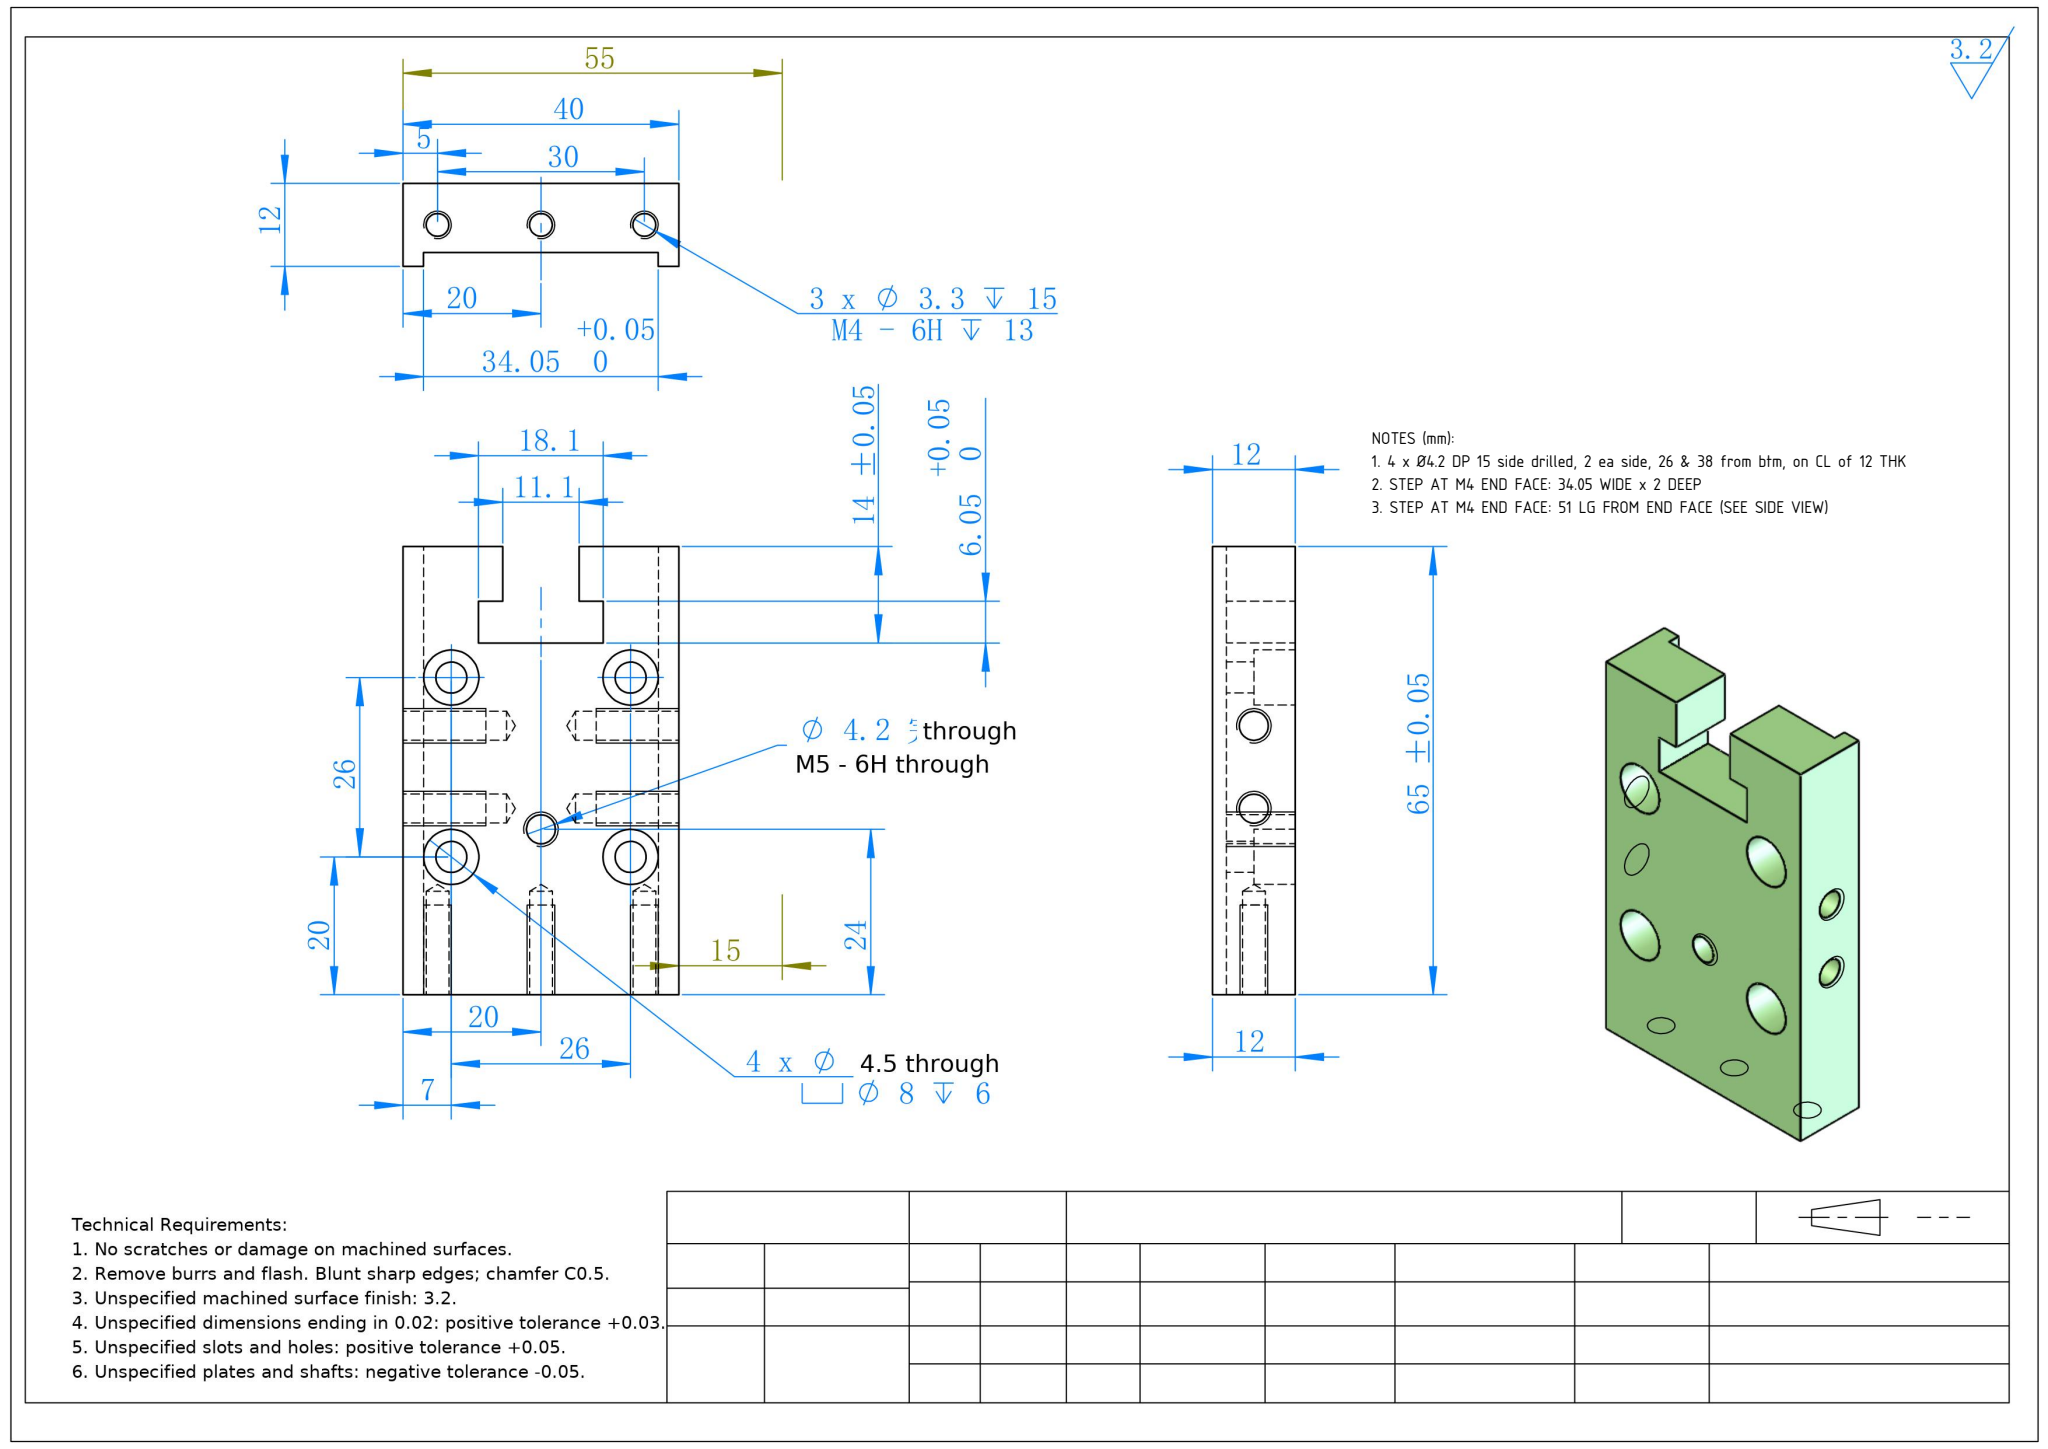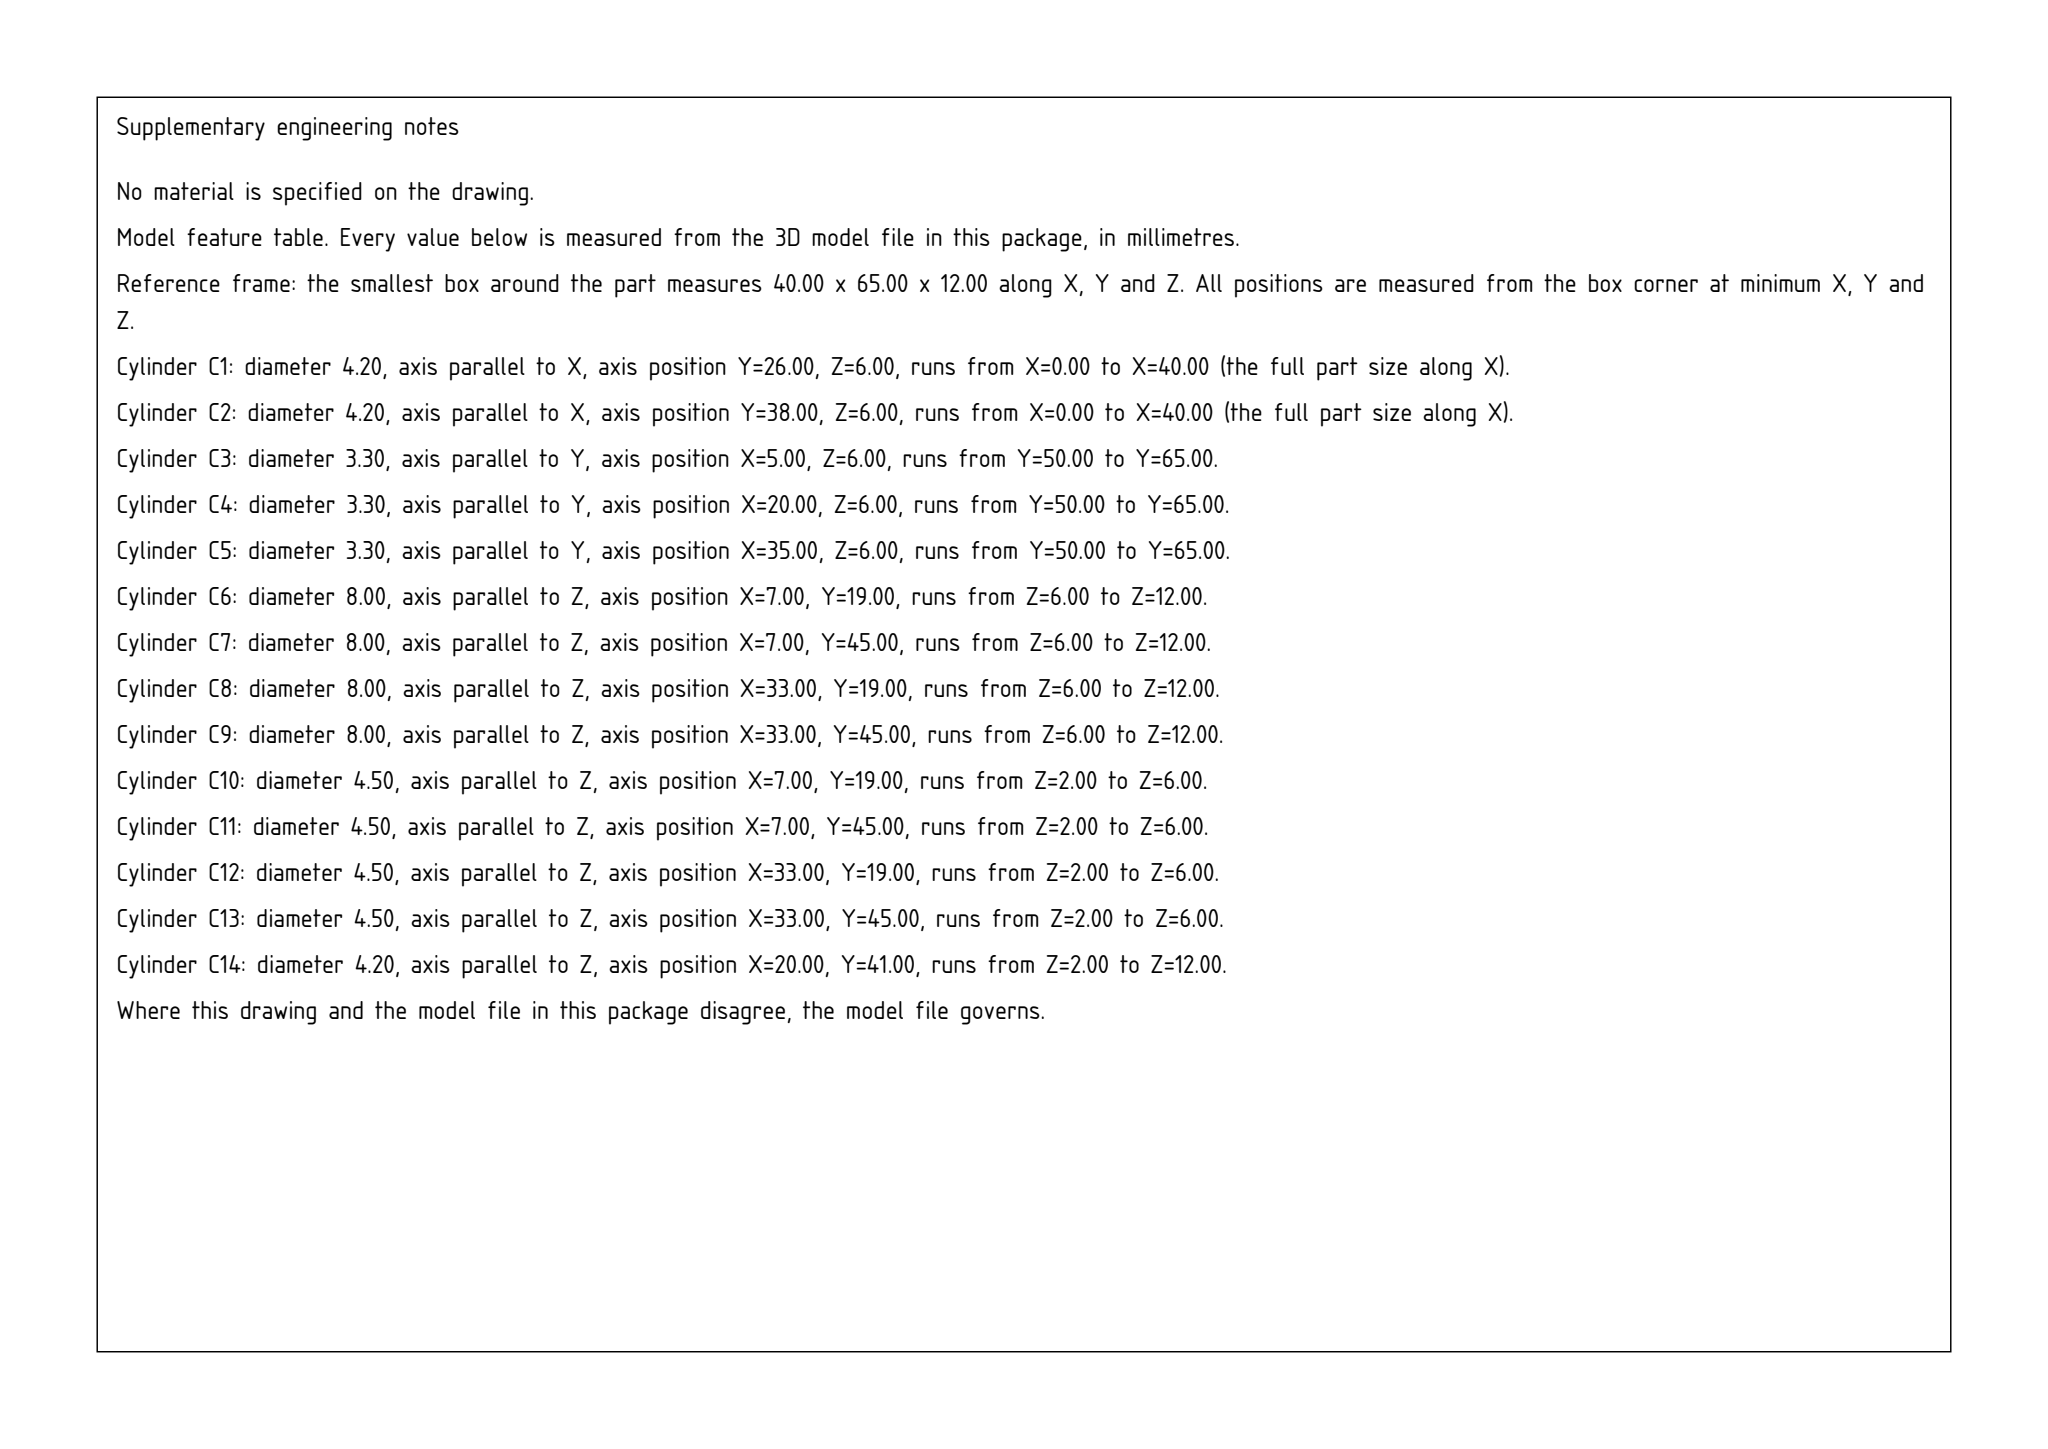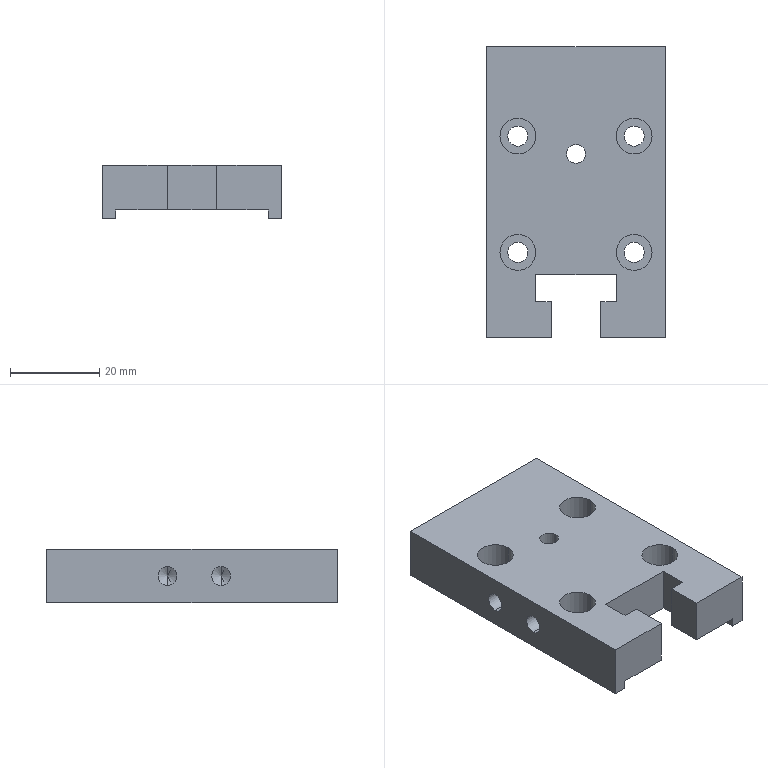Part | SolidWorks | mm | 1 solid | 68 faces | box 40 x 65 x 12 mm | volume 21949 mm3 | cylinder 32 | plane 22 | cone 14 | commonest cylinder face diameters 4.2 x10 8 x8 4.5 x8 3.3 x6
Drawing notes:
4 x Ø4.2 DP 15 side drilled, 2 ea side, 26 & 38 from btm, on CL of 12 THK | from the solid: cylinders [4.2,'x',[null,26.0,6.0],15.0] and [4.2,'x',[null,38.0,6.0],15.0]; z=6.0 is mid of bbox Z=12.0; bbox Y=65 from min corner
STEP AT M4 END FACE: 34.05 WIDE x 2 DEEP | from the solid: Faces x=2.98 & x=37.03 (34.05 wide); relief floor plane z=2.0 vs outer face z=0 -> 2 deep
STEP AT M4 END FACE: 51 LG FROM END FACE (SEE SIDE VIEW) | from the solid: Relief end plane y=14.0 (merged with T-slot bottom), part end y=65.0 -> 65-14=51 long
build123d program:
from build123d import *

# Parameters (mm, degrees)
SKETCH1_W                                       = 40
SKETCH1_H                                       = 65
BOSS_EXTRUDE1_DEPTH                             = 12
CUT_EXTRUDE2_DEPTH                              = 41.003
SKETCH15_W                                      = 34.05
SKETCH15_H                                      = 65
CUT_EXTRUDE4_DEPTH                              = 2
M4_HEX_SOCKET_HEAD_CAP_SCREW_CBORE1_D           = 4.5
M4_HEX_SOCKET_HEAD_CAP_SCREW_CBORE1_CBORE_D     = 8
M4_HEX_SOCKET_HEAD_CAP_SCREW_CBORE1_CBORE_DEPTH = 6
M4_TAPPED_HOLE1_D                               = 3.3
M4_TAPPED_HOLE1_DEPTH                           = 15
M4_TAPPED_HOLE1_TIP                             = 0.9914
M5_TAPPED_HOLE2_D                               = 4.2
M5_TAPPED_HOLE3_AT_2_COUNT                      = 2
M5_TAPPED_HOLE3_AT_2_PITCH                      = 12


with BuildPart() as part:
    # Sketch1 → Boss-Extrude1 (new body)
    with BuildSketch(Plane.XY):
        Rectangle(SKETCH1_W, SKETCH1_H)
    extrude(amount=BOSS_EXTRUDE1_DEPTH)

    # Sketch5 → Cut-Extrude2 (cut, through all)
    with BuildSketch(Plane.XY.offset(12)):
        Polygon((5.55, -24.55), (9.05, -24.55), (9.05, -18.5), (-9.05, -18.5), (-9.05, -24.55), (-5.55, -24.55), (-5.55, -32.5), (5.55, -32.5), align=None)
    extrude(amount=-CUT_EXTRUDE2_DEPTH, mode=Mode.SUBTRACT)

    # Sketch15 → Cut-Extrude4 (cut)
    with BuildSketch(Plane(origin=(0, 0, 0), x_dir=(-1, 0, 0), z_dir=(0, 0, -1))):
        Rectangle(SKETCH15_W, SKETCH15_H)
    extrude(amount=-CUT_EXTRUDE4_DEPTH, mode=Mode.SUBTRACT)

    # M4 Hex Socket Head Cap Screw CBORE1 (through all)
    with Locations(Plane.XY.offset(12)):
        with Locations((-13, -13.5), (13, -13.5), (-13, 12.5), (13, 12.5)):
            CounterBoreHole(M4_HEX_SOCKET_HEAD_CAP_SCREW_CBORE1_D / 2, M4_HEX_SOCKET_HEAD_CAP_SCREW_CBORE1_CBORE_D / 2, M4_HEX_SOCKET_HEAD_CAP_SCREW_CBORE1_CBORE_DEPTH)

    # M4 Tapped Hole1
    with Locations(Plane(origin=(0, 32.5, 0), x_dir=(-1, 0, 0), z_dir=(0, 1, 0))):
        with Locations((15, 6), (0, 6), (-15, 6)):
            Hole(M4_TAPPED_HOLE1_D / 2, depth=M4_TAPPED_HOLE1_DEPTH)
            with Locations((0, 0, -(M4_TAPPED_HOLE1_DEPTH + M4_TAPPED_HOLE1_TIP / 2))):  # 118° drill point
                Cone(0, M4_TAPPED_HOLE1_D / 2, M4_TAPPED_HOLE1_TIP, mode=Mode.SUBTRACT)

    # M5 Tapped Hole2 (through all)
    with Locations(Plane.XY.offset(12)):
        with Locations((0, 8.5)):
            Hole(M5_TAPPED_HOLE2_D / 2)

    # Sketch39 → M5 Tapped Hole3 (revolve, cut)
    with BuildSketch(Plane(origin=(-20, -6.5, 6), x_dir=(0, 0, 1), z_dir=(0, 1, 0))):
        Polygon((0, 0), (0, 16.262), (2.1, 15), (2.1, 0), align=None)
    m5_tapped_hole3 = revolve(axis=Axis((-26.35, -6.5, 6), (1, 0, 0)), mode=Mode.SUBTRACT)

    # M5 Tapped Hole3 at 2: M5 Tapped Hole3 ×2
    with Locations(*[(0, i * M5_TAPPED_HOLE3_AT_2_PITCH, 0) for i in range(1, M5_TAPPED_HOLE3_AT_2_COUNT)]):
        add(m5_tapped_hole3, mode=Mode.SUBTRACT)

    # Mirror1: M5 Tapped Hole3 across plane
    add(m5_tapped_hole3.mirror(Plane(origin=(0, 0, 0), x_dir=(0, 0, 1), z_dir=(1, 0, 0))), mode=Mode.SUBTRACT)

    # Mirror1 copy 1 sketch → Mirror1 copy 1 (revolve, cut)
    with BuildSketch(Plane(origin=(20, 5.5, 6), x_dir=(0, 0, 1), z_dir=(0, 1, 0))):
        Polygon((0, 0), (0, -16.262), (2.1, -15), (2.1, 0), align=None)
    revolve(axis=Axis((26.35, 5.5, 6), (1, 0, 0)), mode=Mode.SUBTRACT)


solid = part.part